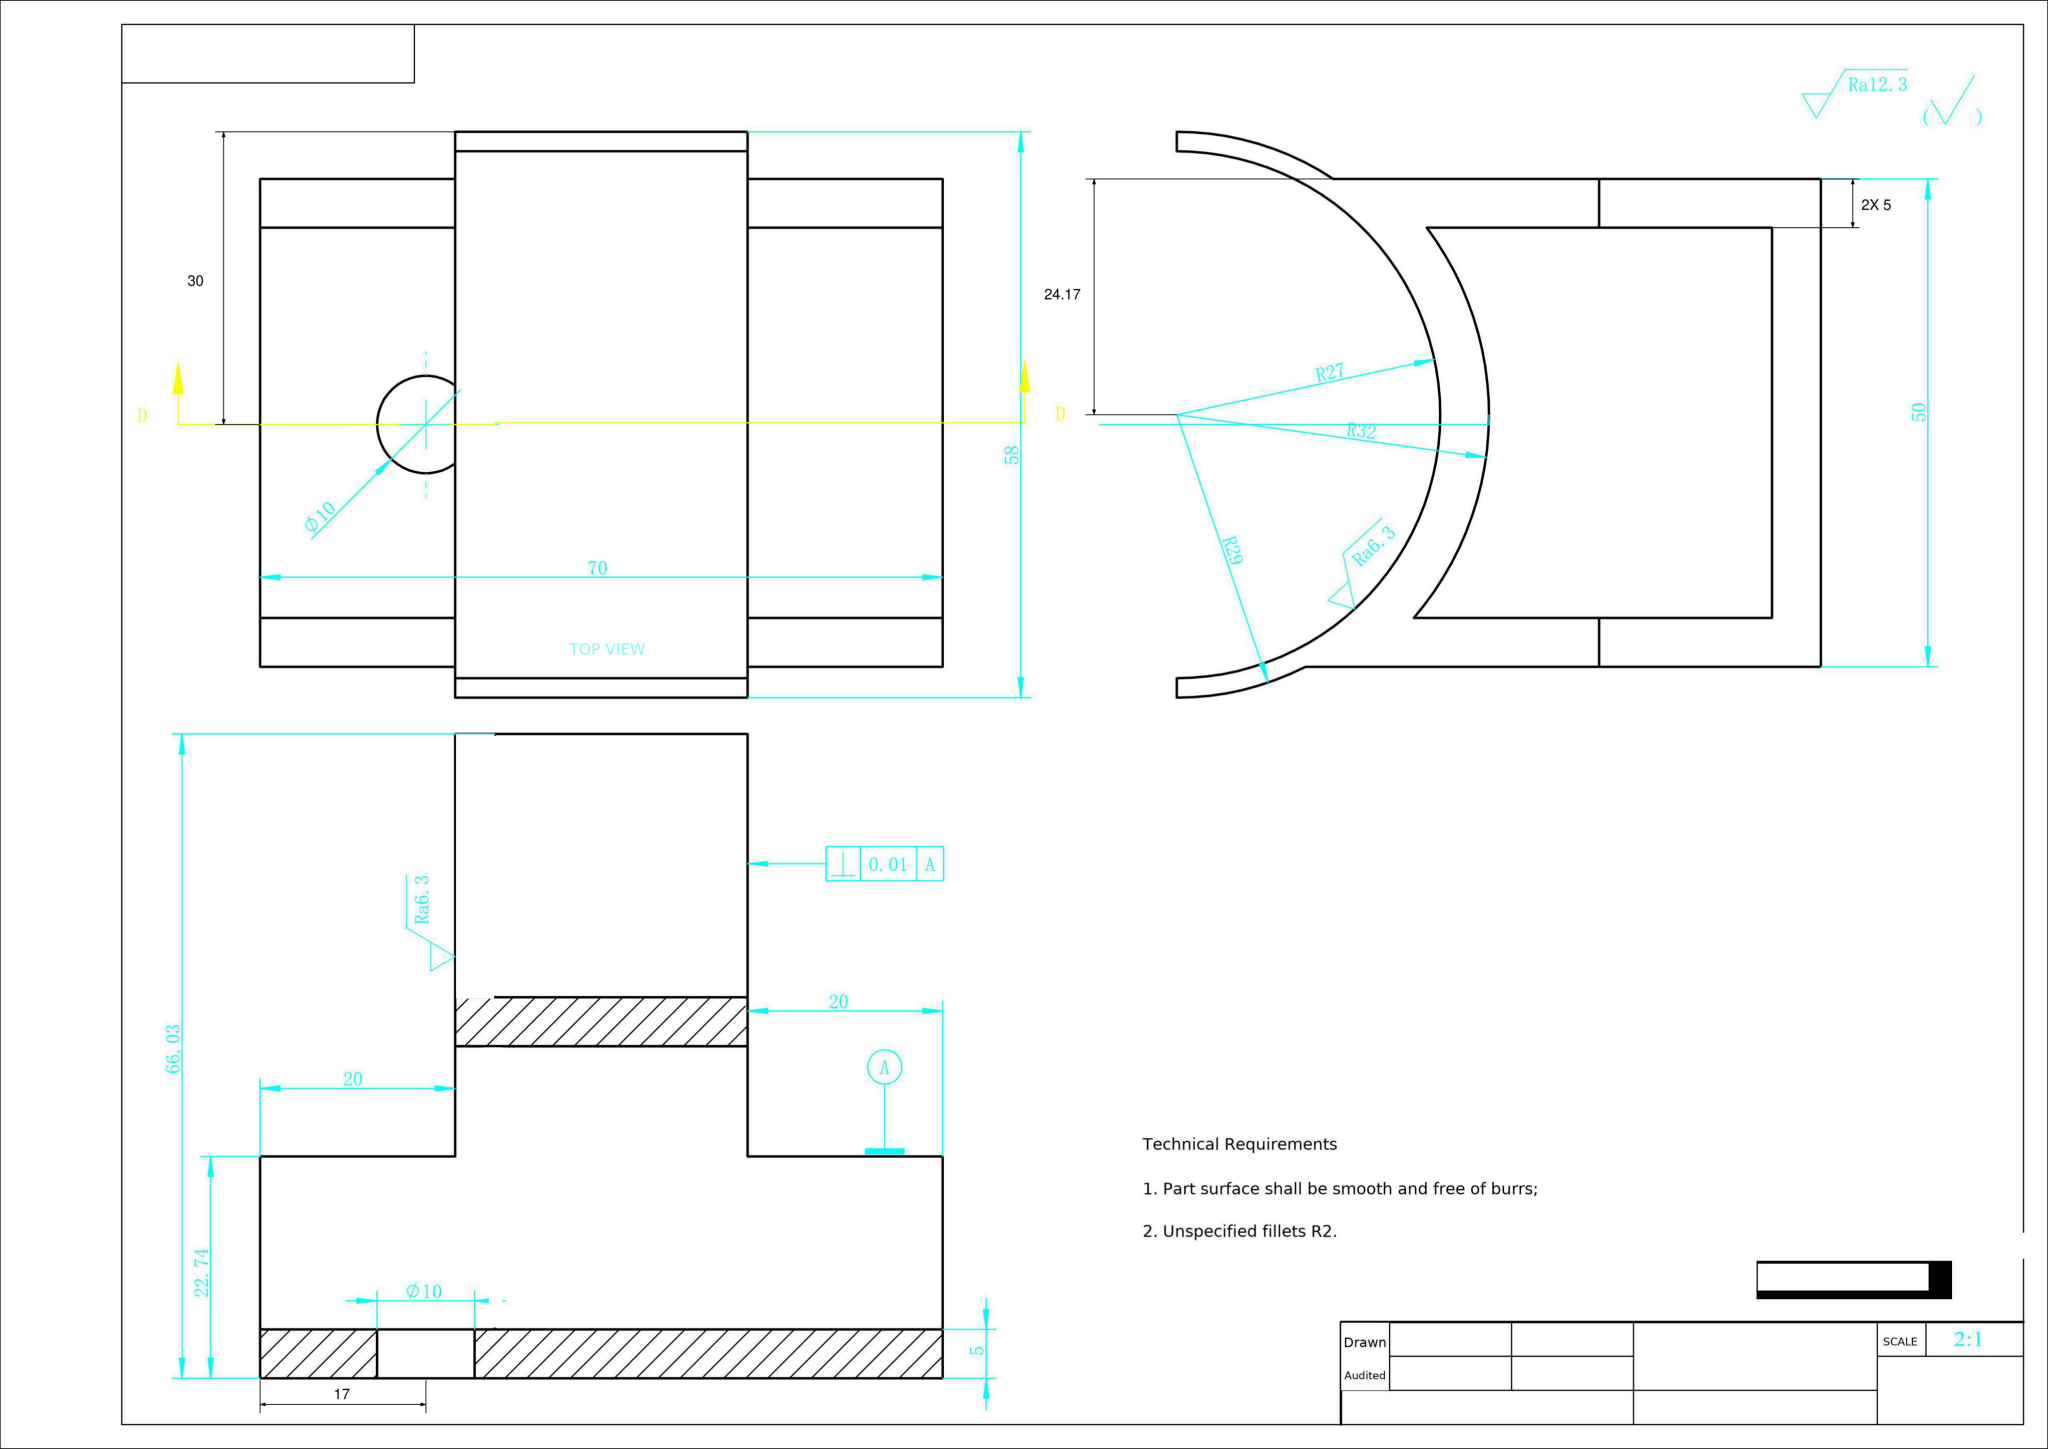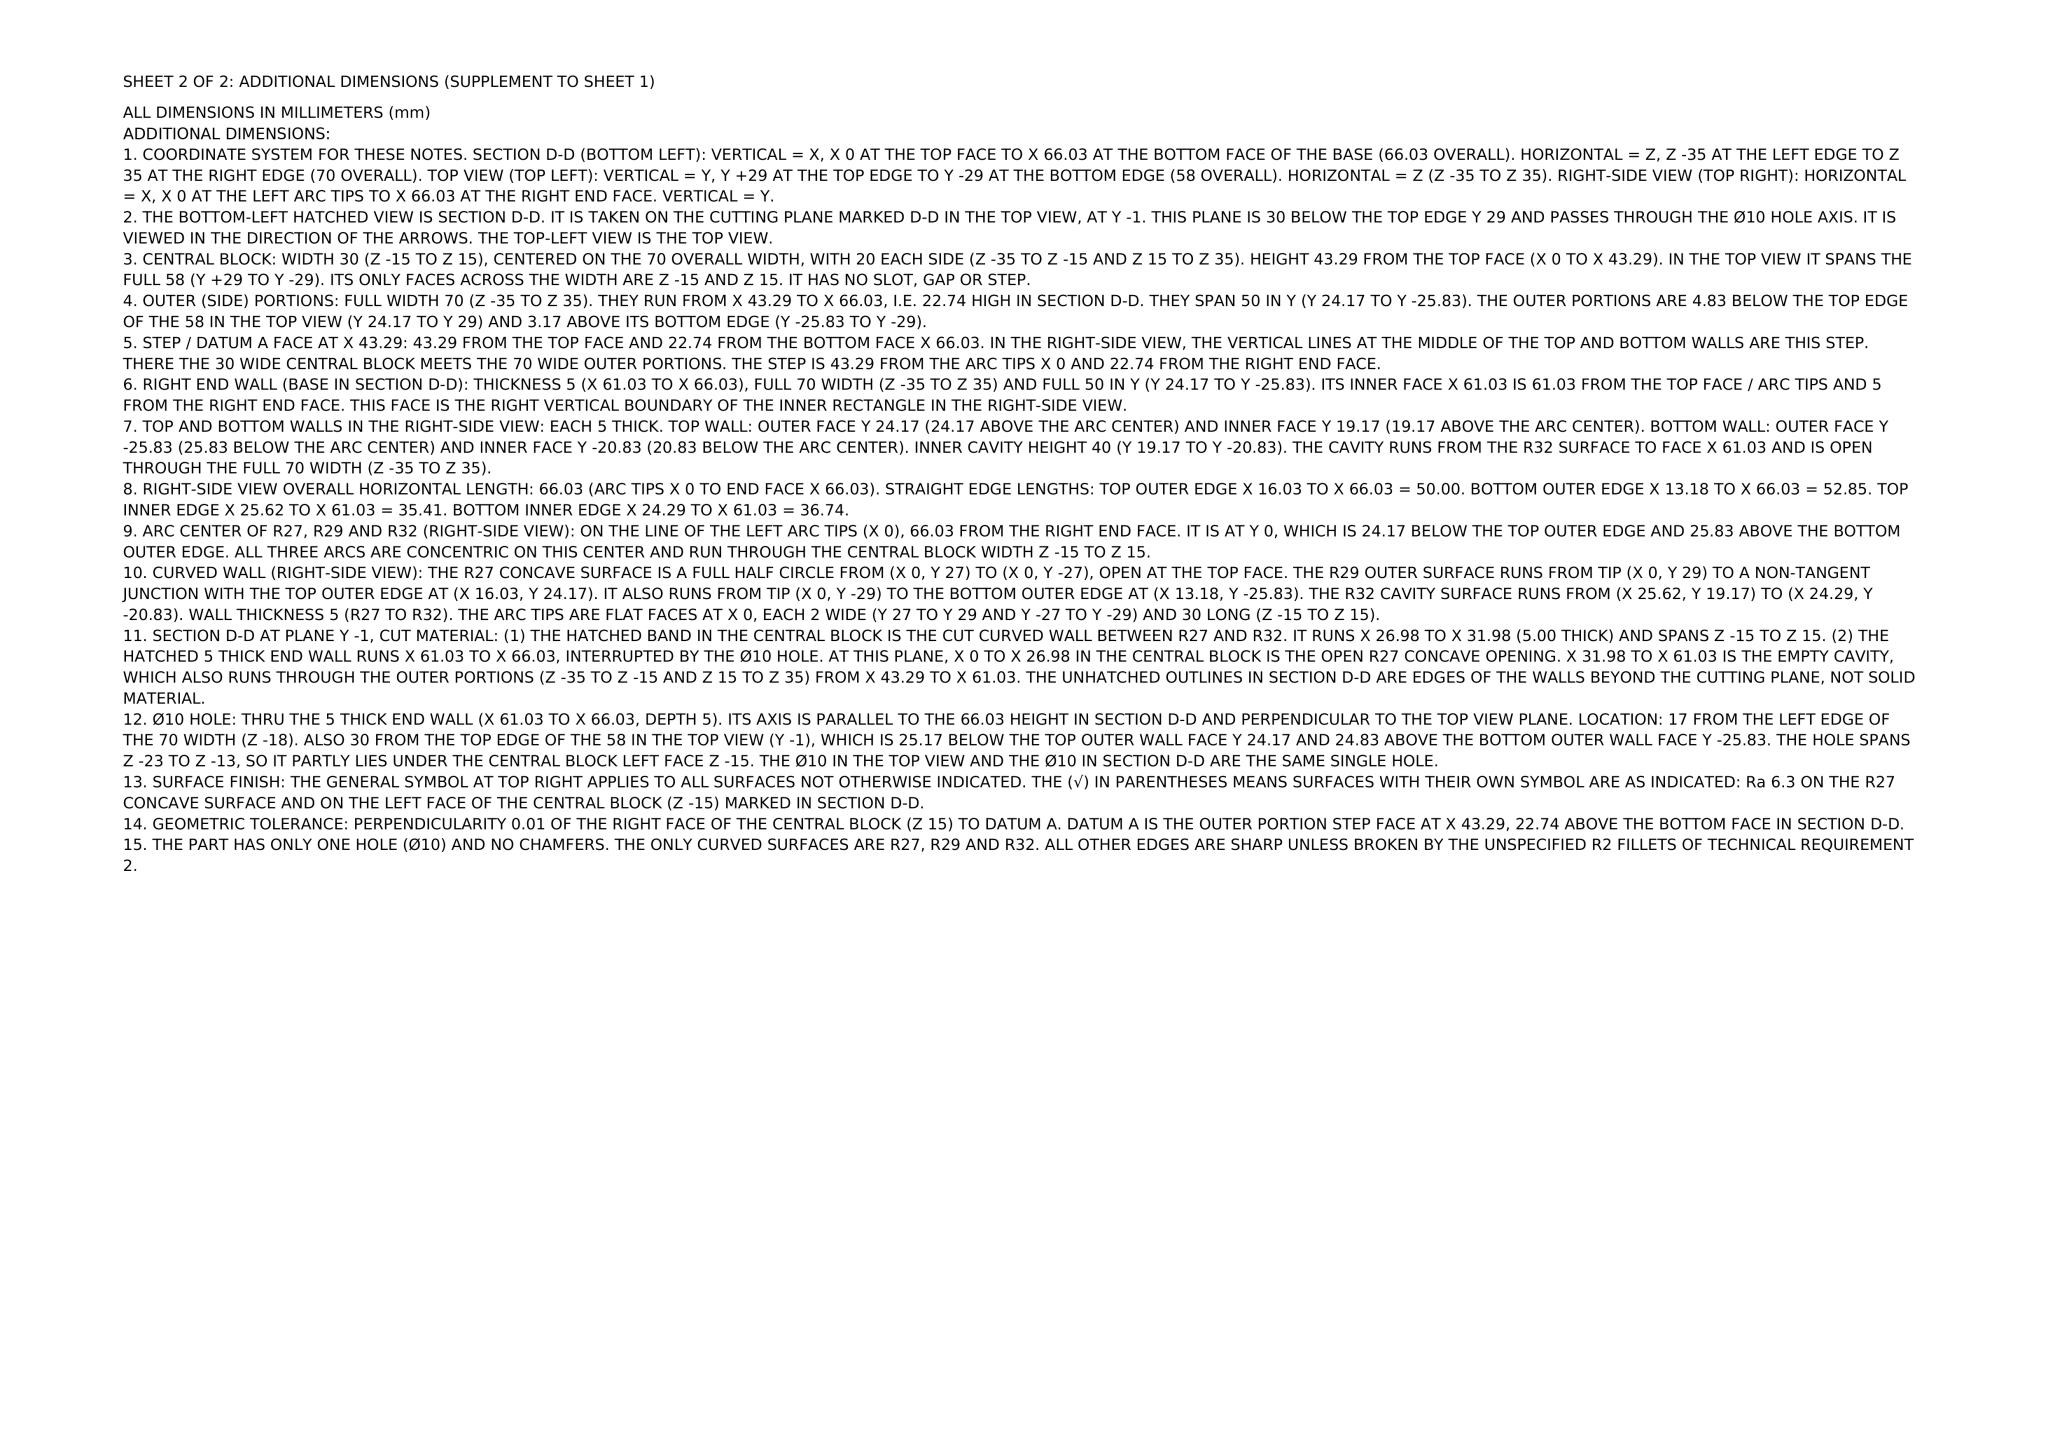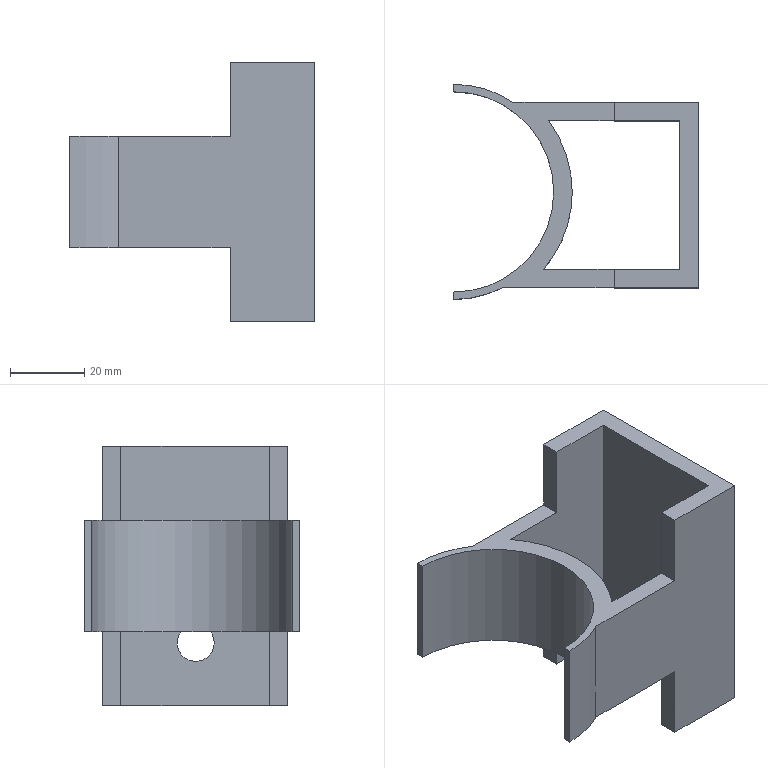Part | NX | mm | 1 solid | 23 faces | box 66.03 x 58 x 70 mm | volume 46292 mm3 | plane 16 | cylinder 7 | commonest cylinder face diameters 10 x2 64 x2 58 x2 54 x1
STEP:
#1=COLOUR_RGB('',0.7765,0.7569,0.7373);
#2=FILL_AREA_STYLE_COLOUR('',#1);
#3=FILL_AREA_STYLE('',(#2));
#4=SURFACE_STYLE_FILL_AREA(#3);
#5=SURFACE_SIDE_STYLE('',(#4));
#6=SURFACE_STYLE_USAGE(.BOTH.,#5);
#7=PRESENTATION_STYLE_ASSIGNMENT((#6));
#8=CARTESIAN_POINT('',(61.03,-6.,-18.));
#9=VERTEX_POINT('',#8);
#10=CARTESIAN_POINT('',(61.03,4.,-18.));
#11=VERTEX_POINT('',#10);
#12=CARTESIAN_POINT('',(61.03,-1.,-18.));
#13=DIRECTION('',(1.,0.,0.));
#14=DIRECTION('',(0.,0.,-1.));
#15=AXIS2_PLACEMENT_3D('',#12,#13,#14);
#16=CIRCLE('',#15,5.);
#17=EDGE_CURVE('',#9,#11,#16,.T.);
#18=ORIENTED_EDGE('',*,*,#17,.F.);
#19=CARTESIAN_POINT('',(66.03,-6.,-18.));
#20=VERTEX_POINT('',#19);
#21=CARTESIAN_POINT('',(56.03,-6.,-18.));
#22=DIRECTION('',(1.,0.,0.));
#23=VECTOR('',#22,1000.);
#24=LINE('',#21,#23);
#25=EDGE_CURVE('',#9,#20,#24,.T.);
#26=ORIENTED_EDGE('',*,*,#25,.T.);
#27=CARTESIAN_POINT('',(66.03,4.,-18.));
#28=VERTEX_POINT('',#27);
#29=CARTESIAN_POINT('',(66.03,-1.,-18.));
#30=DIRECTION('',(1.,0.,0.));
#31=DIRECTION('',(0.,1.,0.));
#32=AXIS2_PLACEMENT_3D('',#29,#30,#31);
#33=CIRCLE('',#32,5.);
#34=EDGE_CURVE('',#20,#28,#33,.T.);
#35=ORIENTED_EDGE('',*,*,#34,.T.);
#36=CARTESIAN_POINT('',(56.03,4.,-18.));
#37=DIRECTION('',(1.,0.,0.));
#38=VECTOR('',#37,1000.);
#39=LINE('',#36,#38);
#40=EDGE_CURVE('',#11,#28,#39,.T.);
#41=ORIENTED_EDGE('',*,*,#40,.F.);
#42=EDGE_LOOP('',(#18,#26,#35,#41));
#43=FACE_OUTER_BOUND('',#42,.T.);
#44=CARTESIAN_POINT('',(56.03,-1.,-18.));
#45=DIRECTION('',(1.,0.,0.));
#46=DIRECTION('',(0.,1.,0.));
#47=AXIS2_PLACEMENT_3D('',#44,#45,#46);
#48=CYLINDRICAL_SURFACE('',#47,5.);
#49=ADVANCED_FACE('',(#43),#48,.F.);
#50=CARTESIAN_POINT('',(24.289,-20.833,-15.));
#51=VERTEX_POINT('',#50);
#52=CARTESIAN_POINT('',(32.,-0.,-15.));
#53=VERTEX_POINT('',#52);
#54=CARTESIAN_POINT('',(0.,0.,-15.));
#55=DIRECTION('',(0.,0.,1.));
#56=DIRECTION('',(1.,0.,-0.));
#57=AXIS2_PLACEMENT_3D('',#54,#55,#56);
#58=CIRCLE('',#57,32.);
#59=EDGE_CURVE('',#51,#53,#58,.T.);
#60=ORIENTED_EDGE('',*,*,#59,.T.);
#61=CARTESIAN_POINT('',(32.,0.,15.));
#62=VERTEX_POINT('',#61);
#63=CARTESIAN_POINT('',(32.,0.,-35.));
#64=DIRECTION('',(0.,0.,1.));
#65=VECTOR('',#64,1000.);
#66=LINE('',#63,#65);
#67=EDGE_CURVE('',#53,#62,#66,.T.);
#68=ORIENTED_EDGE('',*,*,#67,.T.);
#69=CARTESIAN_POINT('',(24.289,-20.833,15.));
#70=VERTEX_POINT('',#69);
#71=CARTESIAN_POINT('',(0.,0.,15.));
#72=DIRECTION('',(-0.,-0.,-1.));
#73=DIRECTION('',(-1.,0.,0.));
#74=AXIS2_PLACEMENT_3D('',#71,#72,#73);
#75=CIRCLE('',#74,32.);
#76=EDGE_CURVE('',#62,#70,#75,.T.);
#77=ORIENTED_EDGE('',*,*,#76,.T.);
#78=CARTESIAN_POINT('',(24.289,-20.833,-35.));
#79=DIRECTION('',(0.,0.,1.));
#80=VECTOR('',#79,1000.);
#81=LINE('',#78,#80);
#82=EDGE_CURVE('',#51,#70,#81,.T.);
#83=ORIENTED_EDGE('',*,*,#82,.F.);
#84=EDGE_LOOP('',(#60,#68,#77,#83));
#85=FACE_OUTER_BOUND('',#84,.T.);
#86=CARTESIAN_POINT('',(0.,0.,-35.));
#87=DIRECTION('',(0.,0.,1.));
#88=DIRECTION('',(1.,0.,0.));
#89=AXIS2_PLACEMENT_3D('',#86,#87,#88);
#90=CYLINDRICAL_SURFACE('',#89,32.);
#91=ADVANCED_FACE('',(#85),#90,.T.);
#92=CARTESIAN_POINT('',(0.,29.,15.));
#93=VERTEX_POINT('',#92);
#94=CARTESIAN_POINT('',(0.,29.,-15.));
#95=VERTEX_POINT('',#94);
#96=CARTESIAN_POINT('',(0.,29.,35.));
#97=DIRECTION('',(0.,0.,-1.));
#98=VECTOR('',#97,1000.);
#99=LINE('',#96,#98);
#100=EDGE_CURVE('',#93,#95,#99,.T.);
#101=ORIENTED_EDGE('',*,*,#100,.F.);
#102=CARTESIAN_POINT('',(16.03,24.167,15.));
#103=VERTEX_POINT('',#102);
#104=CARTESIAN_POINT('',(0.,0.,15.));
#105=DIRECTION('',(-0.,-0.,-1.));
#106=DIRECTION('',(-1.,0.,0.));
#107=AXIS2_PLACEMENT_3D('',#104,#105,#106);
#108=CIRCLE('',#107,29.);
#109=EDGE_CURVE('',#93,#103,#108,.T.);
#110=ORIENTED_EDGE('',*,*,#109,.T.);
#111=CARTESIAN_POINT('',(16.03,24.167,-15.));
#112=VERTEX_POINT('',#111);
#113=CARTESIAN_POINT('',(16.03,24.167,35.));
#114=DIRECTION('',(0.,0.,-1.));
#115=VECTOR('',#114,1000.);
#116=LINE('',#113,#115);
#117=EDGE_CURVE('',#103,#112,#116,.T.);
#118=ORIENTED_EDGE('',*,*,#117,.T.);
#119=CARTESIAN_POINT('',(0.,0.,-15.));
#120=DIRECTION('',(0.,0.,1.));
#121=DIRECTION('',(1.,0.,-0.));
#122=AXIS2_PLACEMENT_3D('',#119,#120,#121);
#123=CIRCLE('',#122,29.);
#124=EDGE_CURVE('',#112,#95,#123,.T.);
#125=ORIENTED_EDGE('',*,*,#124,.T.);
#126=EDGE_LOOP('',(#101,#110,#118,#125));
#127=FACE_OUTER_BOUND('',#126,.T.);
#128=CARTESIAN_POINT('',(0.,0.,35.));
#129=DIRECTION('',(0.,0.,-1.));
#130=DIRECTION('',(-1.,0.,0.));
#131=AXIS2_PLACEMENT_3D('',#128,#129,#130);
#132=CYLINDRICAL_SURFACE('',#131,29.);
#133=ADVANCED_FACE('',(#127),#132,.T.);
#134=CARTESIAN_POINT('',(-0.,27.,15.));
#135=VERTEX_POINT('',#134);
#136=CARTESIAN_POINT('',(-0.,27.,-15.));
#137=VERTEX_POINT('',#136);
#138=CARTESIAN_POINT('',(0.,27.,35.));
#139=DIRECTION('',(0.,0.,-1.));
#140=VECTOR('',#139,1000.);
#141=LINE('',#138,#140);
#142=EDGE_CURVE('',#135,#137,#141,.T.);
#143=ORIENTED_EDGE('',*,*,#142,.F.);
#144=CARTESIAN_POINT('',(0.,29.,15.));
#145=DIRECTION('',(0.,1.,-0.));
#146=VECTOR('',#145,1000.);
#147=LINE('',#144,#146);
#148=EDGE_CURVE('',#135,#93,#147,.T.);
#149=ORIENTED_EDGE('',*,*,#148,.T.);
#150=ORIENTED_EDGE('',*,*,#100,.T.);
#151=CARTESIAN_POINT('',(0.,29.,-15.));
#152=DIRECTION('',(-0.,-1.,0.));
#153=VECTOR('',#152,1000.);
#154=LINE('',#151,#153);
#155=EDGE_CURVE('',#95,#137,#154,.T.);
#156=ORIENTED_EDGE('',*,*,#155,.T.);
#157=EDGE_LOOP('',(#143,#149,#150,#156));
#158=FACE_OUTER_BOUND('',#157,.T.);
#159=CARTESIAN_POINT('',(0.,29.,35.));
#160=DIRECTION('',(1.,-0.,0.));
#161=DIRECTION('',(0.,1.,0.));
#162=AXIS2_PLACEMENT_3D('',#159,#160,#161);
#163=PLANE('',#162);
#164=ADVANCED_FACE('',(#158),#163,.F.);
#165=CARTESIAN_POINT('',(-0.,-27.,15.));
#166=VERTEX_POINT('',#165);
#167=CARTESIAN_POINT('',(0.,-27.,-15.));
#168=VERTEX_POINT('',#167);
#169=CARTESIAN_POINT('',(0.,-27.,35.));
#170=DIRECTION('',(0.,0.,-1.));
#171=VECTOR('',#170,1000.);
#172=LINE('',#169,#171);
#173=EDGE_CURVE('',#166,#168,#172,.T.);
#174=ORIENTED_EDGE('',*,*,#173,.F.);
#175=CARTESIAN_POINT('',(0.,0.,15.));
#176=DIRECTION('',(0.,0.,1.));
#177=DIRECTION('',(-1.,0.,0.));
#178=AXIS2_PLACEMENT_3D('',#175,#176,#177);
#179=CIRCLE('',#178,27.);
#180=EDGE_CURVE('',#166,#135,#179,.T.);
#181=ORIENTED_EDGE('',*,*,#180,.T.);
#182=ORIENTED_EDGE('',*,*,#142,.T.);
#183=CARTESIAN_POINT('',(0.,0.,-15.));
#184=DIRECTION('',(-0.,-0.,-1.));
#185=DIRECTION('',(1.,0.,-0.));
#186=AXIS2_PLACEMENT_3D('',#183,#184,#185);
#187=CIRCLE('',#186,27.);
#188=EDGE_CURVE('',#137,#168,#187,.T.);
#189=ORIENTED_EDGE('',*,*,#188,.T.);
#190=EDGE_LOOP('',(#174,#181,#182,#189));
#191=FACE_OUTER_BOUND('',#190,.T.);
#192=CARTESIAN_POINT('',(0.,0.,35.));
#193=DIRECTION('',(0.,0.,-1.));
#194=DIRECTION('',(-1.,0.,0.));
#195=AXIS2_PLACEMENT_3D('',#192,#193,#194);
#196=CYLINDRICAL_SURFACE('',#195,27.);
#197=ADVANCED_FACE('',(#191),#196,.F.);
#198=CARTESIAN_POINT('',(0.,-29.,15.));
#199=VERTEX_POINT('',#198);
#200=CARTESIAN_POINT('',(0.,-29.,-15.));
#201=VERTEX_POINT('',#200);
#202=CARTESIAN_POINT('',(-0.,-29.,35.));
#203=DIRECTION('',(0.,0.,-1.));
#204=VECTOR('',#203,1000.);
#205=LINE('',#202,#204);
#206=EDGE_CURVE('',#199,#201,#205,.T.);
#207=ORIENTED_EDGE('',*,*,#206,.F.);
#208=CARTESIAN_POINT('',(-0.,-27.,15.));
#209=DIRECTION('',(-0.,1.,0.));
#210=VECTOR('',#209,1000.);
#211=LINE('',#208,#210);
#212=EDGE_CURVE('',#199,#166,#211,.T.);
#213=ORIENTED_EDGE('',*,*,#212,.T.);
#214=ORIENTED_EDGE('',*,*,#173,.T.);
#215=CARTESIAN_POINT('',(-0.,-27.,-15.));
#216=DIRECTION('',(0.,-1.,-0.));
#217=VECTOR('',#216,1000.);
#218=LINE('',#215,#217);
#219=EDGE_CURVE('',#168,#201,#218,.T.);
#220=ORIENTED_EDGE('',*,*,#219,.T.);
#221=EDGE_LOOP('',(#207,#213,#214,#220));
#222=FACE_OUTER_BOUND('',#221,.T.);
#223=CARTESIAN_POINT('',(0.,-27.,35.));
#224=DIRECTION('',(1.,0.,0.));
#225=DIRECTION('',(-0.,1.,0.));
#226=AXIS2_PLACEMENT_3D('',#223,#224,#225);
#227=PLANE('',#226);
#228=ADVANCED_FACE('',(#222),#227,.F.);
#229=CARTESIAN_POINT('',(13.177,-25.833,15.));
#230=VERTEX_POINT('',#229);
#231=CARTESIAN_POINT('',(13.177,-25.833,-15.));
#232=VERTEX_POINT('',#231);
#233=CARTESIAN_POINT('',(13.177,-25.833,35.));
#234=DIRECTION('',(0.,0.,-1.));
#235=VECTOR('',#234,1000.);
#236=LINE('',#233,#235);
#237=EDGE_CURVE('',#230,#232,#236,.T.);
#238=ORIENTED_EDGE('',*,*,#237,.F.);
#239=CARTESIAN_POINT('',(0.,0.,15.));
#240=DIRECTION('',(-0.,-0.,-1.));
#241=DIRECTION('',(-1.,0.,0.));
#242=AXIS2_PLACEMENT_3D('',#239,#240,#241);
#243=CIRCLE('',#242,29.);
#244=EDGE_CURVE('',#230,#199,#243,.T.);
#245=ORIENTED_EDGE('',*,*,#244,.T.);
#246=ORIENTED_EDGE('',*,*,#206,.T.);
#247=CARTESIAN_POINT('',(0.,0.,-15.));
#248=DIRECTION('',(0.,0.,1.));
#249=DIRECTION('',(1.,0.,-0.));
#250=AXIS2_PLACEMENT_3D('',#247,#248,#249);
#251=CIRCLE('',#250,29.);
#252=EDGE_CURVE('',#201,#232,#251,.T.);
#253=ORIENTED_EDGE('',*,*,#252,.T.);
#254=EDGE_LOOP('',(#238,#245,#246,#253));
#255=FACE_OUTER_BOUND('',#254,.T.);
#256=CARTESIAN_POINT('',(0.,0.,35.));
#257=DIRECTION('',(0.,0.,-1.));
#258=DIRECTION('',(-1.,0.,0.));
#259=AXIS2_PLACEMENT_3D('',#256,#257,#258);
#260=CYLINDRICAL_SURFACE('',#259,29.);
#261=ADVANCED_FACE('',(#255),#260,.T.);
#262=CARTESIAN_POINT('',(43.289,-25.833,35.));
#263=VERTEX_POINT('',#262);
#264=CARTESIAN_POINT('',(66.03,-25.833,35.));
#265=VERTEX_POINT('',#264);
#266=CARTESIAN_POINT('',(66.03,-25.833,35.));
#267=DIRECTION('',(1.,0.,0.));
#268=VECTOR('',#267,1000.);
#269=LINE('',#266,#268);
#270=EDGE_CURVE('',#263,#265,#269,.T.);
#271=ORIENTED_EDGE('',*,*,#270,.F.);
#272=CARTESIAN_POINT('',(43.289,-25.833,15.));
#273=VERTEX_POINT('',#272);
#274=CARTESIAN_POINT('',(43.289,-25.833,35.));
#275=DIRECTION('',(0.,0.,-1.));
#276=VECTOR('',#275,1000.);
#277=LINE('',#274,#276);
#278=EDGE_CURVE('',#263,#273,#277,.T.);
#279=ORIENTED_EDGE('',*,*,#278,.T.);
#280=CARTESIAN_POINT('',(66.03,-25.833,15.));
#281=DIRECTION('',(-1.,0.,0.));
#282=VECTOR('',#281,1000.);
#283=LINE('',#280,#282);
#284=EDGE_CURVE('',#273,#230,#283,.T.);
#285=ORIENTED_EDGE('',*,*,#284,.T.);
#286=ORIENTED_EDGE('',*,*,#237,.T.);
#287=CARTESIAN_POINT('',(43.289,-25.833,-15.));
#288=VERTEX_POINT('',#287);
#289=CARTESIAN_POINT('',(66.03,-25.833,-15.));
#290=DIRECTION('',(1.,0.,-0.));
#291=VECTOR('',#290,1000.);
#292=LINE('',#289,#291);
#293=EDGE_CURVE('',#232,#288,#292,.T.);
#294=ORIENTED_EDGE('',*,*,#293,.T.);
#295=CARTESIAN_POINT('',(43.289,-25.833,-35.));
#296=VERTEX_POINT('',#295);
#297=CARTESIAN_POINT('',(43.289,-25.833,35.));
#298=DIRECTION('',(0.,0.,-1.));
#299=VECTOR('',#298,1000.);
#300=LINE('',#297,#299);
#301=EDGE_CURVE('',#288,#296,#300,.T.);
#302=ORIENTED_EDGE('',*,*,#301,.T.);
#303=CARTESIAN_POINT('',(66.03,-25.833,-35.));
#304=VERTEX_POINT('',#303);
#305=CARTESIAN_POINT('',(66.03,-25.833,-35.));
#306=DIRECTION('',(1.,0.,0.));
#307=VECTOR('',#306,1000.);
#308=LINE('',#305,#307);
#309=EDGE_CURVE('',#296,#304,#308,.T.);
#310=ORIENTED_EDGE('',*,*,#309,.T.);
#311=CARTESIAN_POINT('',(66.03,-25.833,35.));
#312=DIRECTION('',(0.,0.,-1.));
#313=VECTOR('',#312,1000.);
#314=LINE('',#311,#313);
#315=EDGE_CURVE('',#265,#304,#314,.T.);
#316=ORIENTED_EDGE('',*,*,#315,.F.);
#317=EDGE_LOOP('',(#271,#279,#285,#286,#294,#302,#310,#316));
#318=FACE_OUTER_BOUND('',#317,.T.);
#319=CARTESIAN_POINT('',(66.03,-25.833,35.));
#320=DIRECTION('',(0.,1.,0.));
#321=DIRECTION('',(0.,0.,1.));
#322=AXIS2_PLACEMENT_3D('',#319,#320,#321);
#323=PLANE('',#322);
#324=ADVANCED_FACE('',(#318),#323,.F.);
#325=CARTESIAN_POINT('',(66.03,-1.,-18.));
#326=DIRECTION('',(1.,0.,0.));
#327=DIRECTION('',(0.,1.,0.));
#328=AXIS2_PLACEMENT_3D('',#325,#326,#327);
#329=CIRCLE('',#328,5.);
#330=EDGE_CURVE('',#28,#20,#329,.T.);
#331=ORIENTED_EDGE('',*,*,#330,.F.);
#332=ORIENTED_EDGE('',*,*,#34,.F.);
#333=EDGE_LOOP('',(#331,#332));
#334=FACE_BOUND('',#333,.T.);
#335=CARTESIAN_POINT('',(66.03,24.167,-35.));
#336=VERTEX_POINT('',#335);
#337=CARTESIAN_POINT('',(66.03,-25.833,-35.));
#338=DIRECTION('',(-0.,1.,0.));
#339=VECTOR('',#338,1000.);
#340=LINE('',#337,#339);
#341=EDGE_CURVE('',#304,#336,#340,.T.);
#342=ORIENTED_EDGE('',*,*,#341,.T.);
#343=CARTESIAN_POINT('',(66.03,24.167,35.));
#344=VERTEX_POINT('',#343);
#345=CARTESIAN_POINT('',(66.03,24.167,35.));
#346=DIRECTION('',(0.,0.,-1.));
#347=VECTOR('',#346,1000.);
#348=LINE('',#345,#347);
#349=EDGE_CURVE('',#344,#336,#348,.T.);
#350=ORIENTED_EDGE('',*,*,#349,.F.);
#351=CARTESIAN_POINT('',(66.03,-25.833,35.));
#352=DIRECTION('',(-0.,1.,0.));
#353=VECTOR('',#352,1000.);
#354=LINE('',#351,#353);
#355=EDGE_CURVE('',#265,#344,#354,.T.);
#356=ORIENTED_EDGE('',*,*,#355,.F.);
#357=ORIENTED_EDGE('',*,*,#315,.T.);
#358=EDGE_LOOP('',(#342,#350,#356,#357));
#359=FACE_OUTER_BOUND('',#358,.T.);
#360=CARTESIAN_POINT('',(66.03,-25.833,35.));
#361=DIRECTION('',(-1.,-0.,0.));
#362=DIRECTION('',(0.,-1.,0.));
#363=AXIS2_PLACEMENT_3D('',#360,#361,#362);
#364=PLANE('',#363);
#365=ADVANCED_FACE('',(#334,#359),#364,.F.);
#366=CARTESIAN_POINT('',(43.289,24.167,15.));
#367=VERTEX_POINT('',#366);
#368=CARTESIAN_POINT('',(66.03,24.167,15.));
#369=DIRECTION('',(1.,0.,-0.));
#370=VECTOR('',#369,1000.);
#371=LINE('',#368,#370);
#372=EDGE_CURVE('',#103,#367,#371,.T.);
#373=ORIENTED_EDGE('',*,*,#372,.T.);
#374=CARTESIAN_POINT('',(43.289,24.167,35.));
#375=VERTEX_POINT('',#374);
#376=CARTESIAN_POINT('',(43.289,24.167,35.));
#377=DIRECTION('',(0.,0.,1.));
#378=VECTOR('',#377,1000.);
#379=LINE('',#376,#378);
#380=EDGE_CURVE('',#367,#375,#379,.T.);
#381=ORIENTED_EDGE('',*,*,#380,.T.);
#382=CARTESIAN_POINT('',(66.03,24.167,35.));
#383=DIRECTION('',(-1.,-0.,0.));
#384=VECTOR('',#383,1000.);
#385=LINE('',#382,#384);
#386=EDGE_CURVE('',#344,#375,#385,.T.);
#387=ORIENTED_EDGE('',*,*,#386,.F.);
#388=ORIENTED_EDGE('',*,*,#349,.T.);
#389=CARTESIAN_POINT('',(43.289,24.167,-35.));
#390=VERTEX_POINT('',#389);
#391=CARTESIAN_POINT('',(66.03,24.167,-35.));
#392=DIRECTION('',(-1.,-0.,0.));
#393=VECTOR('',#392,1000.);
#394=LINE('',#391,#393);
#395=EDGE_CURVE('',#336,#390,#394,.T.);
#396=ORIENTED_EDGE('',*,*,#395,.T.);
#397=CARTESIAN_POINT('',(43.289,24.167,-15.));
#398=VERTEX_POINT('',#397);
#399=CARTESIAN_POINT('',(43.289,24.167,35.));
#400=DIRECTION('',(0.,0.,1.));
#401=VECTOR('',#400,1000.);
#402=LINE('',#399,#401);
#403=EDGE_CURVE('',#390,#398,#402,.T.);
#404=ORIENTED_EDGE('',*,*,#403,.T.);
#405=CARTESIAN_POINT('',(66.03,24.167,-15.));
#406=DIRECTION('',(-1.,-0.,0.));
#407=VECTOR('',#406,1000.);
#408=LINE('',#405,#407);
#409=EDGE_CURVE('',#398,#112,#408,.T.);
#410=ORIENTED_EDGE('',*,*,#409,.T.);
#411=ORIENTED_EDGE('',*,*,#117,.F.);
#412=EDGE_LOOP('',(#373,#381,#387,#388,#396,#404,#410,#411));
#413=FACE_OUTER_BOUND('',#412,.T.);
#414=CARTESIAN_POINT('',(66.03,24.167,35.));
#415=DIRECTION('',(0.,-1.,0.));
#416=DIRECTION('',(1.,0.,0.));
#417=AXIS2_PLACEMENT_3D('',#414,#415,#416);
#418=PLANE('',#417);
#419=ADVANCED_FACE('',(#413),#418,.F.);
#420=CARTESIAN_POINT('',(43.289,-20.833,35.));
#421=VERTEX_POINT('',#420);
#422=CARTESIAN_POINT('',(43.289,0.,35.));
#423=DIRECTION('',(-0.,1.,0.));
#424=VECTOR('',#423,1000.);
#425=LINE('',#422,#424);
#426=EDGE_CURVE('',#263,#421,#425,.T.);
#427=ORIENTED_EDGE('',*,*,#426,.F.);
#428=ORIENTED_EDGE('',*,*,#270,.T.);
#429=ORIENTED_EDGE('',*,*,#355,.T.);
#430=ORIENTED_EDGE('',*,*,#386,.T.);
#431=CARTESIAN_POINT('',(43.289,19.167,35.));
#432=VERTEX_POINT('',#431);
#433=CARTESIAN_POINT('',(43.289,0.,35.));
#434=DIRECTION('',(-0.,1.,0.));
#435=VECTOR('',#434,1000.);
#436=LINE('',#433,#435);
#437=EDGE_CURVE('',#432,#375,#436,.T.);
#438=ORIENTED_EDGE('',*,*,#437,.F.);
#439=CARTESIAN_POINT('',(61.03,19.167,35.));
#440=VERTEX_POINT('',#439);
#441=CARTESIAN_POINT('',(61.03,19.167,35.));
#442=DIRECTION('',(-1.,0.,0.));
#443=VECTOR('',#442,1000.);
#444=LINE('',#441,#443);
#445=EDGE_CURVE('',#440,#432,#444,.T.);
#446=ORIENTED_EDGE('',*,*,#445,.F.);
#447=CARTESIAN_POINT('',(61.03,-20.833,35.));
#448=VERTEX_POINT('',#447);
#449=CARTESIAN_POINT('',(61.03,-20.833,35.));
#450=DIRECTION('',(0.,1.,0.));
#451=VECTOR('',#450,1000.);
#452=LINE('',#449,#451);
#453=EDGE_CURVE('',#448,#440,#452,.T.);
#454=ORIENTED_EDGE('',*,*,#453,.F.);
#455=CARTESIAN_POINT('',(24.289,-20.833,35.));
#456=DIRECTION('',(1.,0.,0.));
#457=VECTOR('',#456,1000.);
#458=LINE('',#455,#457);
#459=EDGE_CURVE('',#421,#448,#458,.T.);
#460=ORIENTED_EDGE('',*,*,#459,.F.);
#461=EDGE_LOOP('',(#427,#428,#429,#430,#438,#446,#454,#460));
#462=FACE_OUTER_BOUND('',#461,.T.);
#463=CARTESIAN_POINT('',(0.,0.,35.));
#464=DIRECTION('',(0.,0.,1.));
#465=DIRECTION('',(1.,0.,0.));
#466=AXIS2_PLACEMENT_3D('',#463,#464,#465);
#467=PLANE('',#466);
#468=ADVANCED_FACE('',(#462),#467,.T.);
#469=ORIENTED_EDGE('',*,*,#309,.F.);
#470=CARTESIAN_POINT('',(43.289,-20.833,-35.));
#471=VERTEX_POINT('',#470);
#472=CARTESIAN_POINT('',(43.289,0.,-35.));
#473=DIRECTION('',(-0.,1.,0.));
#474=VECTOR('',#473,1000.);
#475=LINE('',#472,#474);
#476=EDGE_CURVE('',#296,#471,#475,.T.);
#477=ORIENTED_EDGE('',*,*,#476,.T.);
#478=CARTESIAN_POINT('',(61.03,-20.833,-35.));
#479=VERTEX_POINT('',#478);
#480=CARTESIAN_POINT('',(24.289,-20.833,-35.));
#481=DIRECTION('',(1.,0.,0.));
#482=VECTOR('',#481,1000.);
#483=LINE('',#480,#482);
#484=EDGE_CURVE('',#471,#479,#483,.T.);
#485=ORIENTED_EDGE('',*,*,#484,.T.);
#486=CARTESIAN_POINT('',(61.03,19.167,-35.));
#487=VERTEX_POINT('',#486);
#488=CARTESIAN_POINT('',(61.03,-20.833,-35.));
#489=DIRECTION('',(0.,1.,0.));
#490=VECTOR('',#489,1000.);
#491=LINE('',#488,#490);
#492=EDGE_CURVE('',#479,#487,#491,.T.);
#493=ORIENTED_EDGE('',*,*,#492,.T.);
#494=CARTESIAN_POINT('',(43.289,19.167,-35.));
#495=VERTEX_POINT('',#494);
#496=CARTESIAN_POINT('',(61.03,19.167,-35.));
#497=DIRECTION('',(-1.,0.,0.));
#498=VECTOR('',#497,1000.);
#499=LINE('',#496,#498);
#500=EDGE_CURVE('',#487,#495,#499,.T.);
#501=ORIENTED_EDGE('',*,*,#500,.T.);
#502=CARTESIAN_POINT('',(43.289,0.,-35.));
#503=DIRECTION('',(-0.,1.,0.));
#504=VECTOR('',#503,1000.);
#505=LINE('',#502,#504);
#506=EDGE_CURVE('',#495,#390,#505,.T.);
#507=ORIENTED_EDGE('',*,*,#506,.T.);
#508=ORIENTED_EDGE('',*,*,#395,.F.);
#509=ORIENTED_EDGE('',*,*,#341,.F.);
#510=EDGE_LOOP('',(#469,#477,#485,#493,#501,#507,#508,#509));
#511=FACE_OUTER_BOUND('',#510,.T.);
#512=CARTESIAN_POINT('',(0.,0.,-35.));
#513=DIRECTION('',(0.,0.,1.));
#514=DIRECTION('',(1.,0.,0.));
#515=AXIS2_PLACEMENT_3D('',#512,#513,#514);
#516=PLANE('',#515);
#517=ADVANCED_FACE('',(#511),#516,.F.);
#518=CARTESIAN_POINT('',(61.03,-1.,-18.));
#519=DIRECTION('',(1.,0.,0.));
#520=DIRECTION('',(0.,0.,-1.));
#521=AXIS2_PLACEMENT_3D('',#518,#519,#520);
#522=CIRCLE('',#521,5.);
#523=EDGE_CURVE('',#11,#9,#522,.T.);
#524=ORIENTED_EDGE('',*,*,#523,.T.);
#525=ORIENTED_EDGE('',*,*,#17,.T.);
#526=EDGE_LOOP('',(#524,#525));
#527=FACE_BOUND('',#526,.T.);
#528=ORIENTED_EDGE('',*,*,#453,.T.);
#529=CARTESIAN_POINT('',(61.03,19.167,-35.));
#530=DIRECTION('',(0.,0.,1.));
#531=VECTOR('',#530,1000.);
#532=LINE('',#529,#531);
#533=EDGE_CURVE('',#487,#440,#532,.T.);
#534=ORIENTED_EDGE('',*,*,#533,.F.);
#535=ORIENTED_EDGE('',*,*,#492,.F.);
#536=CARTESIAN_POINT('',(61.03,-20.833,-35.));
#537=DIRECTION('',(0.,0.,1.));
#538=VECTOR('',#537,1000.);
#539=LINE('',#536,#538);
#540=EDGE_CURVE('',#479,#448,#539,.T.);
#541=ORIENTED_EDGE('',*,*,#540,.T.);
#542=EDGE_LOOP('',(#528,#534,#535,#541));
#543=FACE_OUTER_BOUND('',#542,.T.);
#544=CARTESIAN_POINT('',(61.03,-20.833,-35.));
#545=DIRECTION('',(1.,0.,0.));
#546=DIRECTION('',(0.,0.,-1.));
#547=AXIS2_PLACEMENT_3D('',#544,#545,#546);
#548=PLANE('',#547);
#549=ADVANCED_FACE('',(#527,#543),#548,.F.);
#550=CARTESIAN_POINT('',(43.289,-20.833,15.));
#551=VERTEX_POINT('',#550);
#552=CARTESIAN_POINT('',(24.289,-20.833,15.));
#553=DIRECTION('',(1.,0.,-0.));
#554=VECTOR('',#553,1000.);
#555=LINE('',#552,#554);
#556=EDGE_CURVE('',#70,#551,#555,.T.);
#557=ORIENTED_EDGE('',*,*,#556,.T.);
#558=CARTESIAN_POINT('',(43.289,-20.833,-35.));
#559=DIRECTION('',(0.,0.,1.));
#560=VECTOR('',#559,1000.);
#561=LINE('',#558,#560);
#562=EDGE_CURVE('',#551,#421,#561,.T.);
#563=ORIENTED_EDGE('',*,*,#562,.T.);
#564=ORIENTED_EDGE('',*,*,#459,.T.);
#565=ORIENTED_EDGE('',*,*,#540,.F.);
#566=ORIENTED_EDGE('',*,*,#484,.F.);
#567=CARTESIAN_POINT('',(43.289,-20.833,-15.));
#568=VERTEX_POINT('',#567);
#569=CARTESIAN_POINT('',(43.289,-20.833,-35.));
#570=DIRECTION('',(0.,0.,1.));
#571=VECTOR('',#570,1000.);
#572=LINE('',#569,#571);
#573=EDGE_CURVE('',#471,#568,#572,.T.);
#574=ORIENTED_EDGE('',*,*,#573,.T.);
#575=CARTESIAN_POINT('',(24.289,-20.833,-15.));
#576=DIRECTION('',(-1.,0.,0.));
#577=VECTOR('',#576,1000.);
#578=LINE('',#575,#577);
#579=EDGE_CURVE('',#568,#51,#578,.T.);
#580=ORIENTED_EDGE('',*,*,#579,.T.);
#581=ORIENTED_EDGE('',*,*,#82,.T.);
#582=EDGE_LOOP('',(#557,#563,#564,#565,#566,#574,#580,#581));
#583=FACE_OUTER_BOUND('',#582,.T.);
#584=CARTESIAN_POINT('',(24.289,-20.833,-35.));
#585=DIRECTION('',(0.,-1.,0.));
#586=DIRECTION('',(0.,0.,-1.));
#587=AXIS2_PLACEMENT_3D('',#584,#585,#586);
#588=PLANE('',#587);
#589=ADVANCED_FACE('',(#583),#588,.F.);
#590=ORIENTED_EDGE('',*,*,#67,.F.);
#591=CARTESIAN_POINT('',(25.625,19.167,-15.));
#592=VERTEX_POINT('',#591);
#593=CARTESIAN_POINT('',(0.,0.,-15.));
#594=DIRECTION('',(0.,0.,1.));
#595=DIRECTION('',(1.,0.,-0.));
#596=AXIS2_PLACEMENT_3D('',#593,#594,#595);
#597=CIRCLE('',#596,32.);
#598=EDGE_CURVE('',#53,#592,#597,.T.);
#599=ORIENTED_EDGE('',*,*,#598,.T.);
#600=CARTESIAN_POINT('',(25.625,19.167,15.));
#601=VERTEX_POINT('',#600);
#602=CARTESIAN_POINT('',(25.625,19.167,-35.));
#603=DIRECTION('',(0.,0.,1.));
#604=VECTOR('',#603,1000.);
#605=LINE('',#602,#604);
#606=EDGE_CURVE('',#592,#601,#605,.T.);
#607=ORIENTED_EDGE('',*,*,#606,.T.);
#608=CARTESIAN_POINT('',(0.,0.,15.));
#609=DIRECTION('',(-0.,-0.,-1.));
#610=DIRECTION('',(-1.,0.,0.));
#611=AXIS2_PLACEMENT_3D('',#608,#609,#610);
#612=CIRCLE('',#611,32.);
#613=EDGE_CURVE('',#601,#62,#612,.T.);
#614=ORIENTED_EDGE('',*,*,#613,.T.);
#615=EDGE_LOOP('',(#590,#599,#607,#614));
#616=FACE_OUTER_BOUND('',#615,.T.);
#617=CARTESIAN_POINT('',(0.,0.,-35.));
#618=DIRECTION('',(0.,0.,1.));
#619=DIRECTION('',(1.,0.,0.));
#620=AXIS2_PLACEMENT_3D('',#617,#618,#619);
#621=CYLINDRICAL_SURFACE('',#620,32.);
#622=ADVANCED_FACE('',(#616),#621,.T.);
#623=ORIENTED_EDGE('',*,*,#445,.T.);
#624=CARTESIAN_POINT('',(43.289,19.167,15.));
#625=VERTEX_POINT('',#624);
#626=CARTESIAN_POINT('',(43.289,19.167,-35.));
#627=DIRECTION('',(0.,0.,-1.));
#628=VECTOR('',#627,1000.);
#629=LINE('',#626,#628);
#630=EDGE_CURVE('',#432,#625,#629,.T.);
#631=ORIENTED_EDGE('',*,*,#630,.T.);
#632=CARTESIAN_POINT('',(61.03,19.167,15.));
#633=DIRECTION('',(-1.,0.,0.));
#634=VECTOR('',#633,1000.);
#635=LINE('',#632,#634);
#636=EDGE_CURVE('',#625,#601,#635,.T.);
#637=ORIENTED_EDGE('',*,*,#636,.T.);
#638=ORIENTED_EDGE('',*,*,#606,.F.);
#639=CARTESIAN_POINT('',(43.289,19.167,-15.));
#640=VERTEX_POINT('',#639);
#641=CARTESIAN_POINT('',(61.03,19.167,-15.));
#642=DIRECTION('',(1.,0.,-0.));
#643=VECTOR('',#642,1000.);
#644=LINE('',#641,#643);
#645=EDGE_CURVE('',#592,#640,#644,.T.);
#646=ORIENTED_EDGE('',*,*,#645,.T.);
#647=CARTESIAN_POINT('',(43.289,19.167,-35.));
#648=DIRECTION('',(0.,0.,-1.));
#649=VECTOR('',#648,1000.);
#650=LINE('',#647,#649);
#651=EDGE_CURVE('',#640,#495,#650,.T.);
#652=ORIENTED_EDGE('',*,*,#651,.T.);
#653=ORIENTED_EDGE('',*,*,#500,.F.);
#654=ORIENTED_EDGE('',*,*,#533,.T.);
#655=EDGE_LOOP('',(#623,#631,#637,#638,#646,#652,#653,#654));
#656=FACE_OUTER_BOUND('',#655,.T.);
#657=CARTESIAN_POINT('',(61.03,19.167,-35.));
#658=DIRECTION('',(0.,1.,0.));
#659=DIRECTION('',(0.,0.,1.));
#660=AXIS2_PLACEMENT_3D('',#657,#658,#659);
#661=PLANE('',#660);
#662=ADVANCED_FACE('',(#656),#661,.F.);
#663=ORIENTED_EDGE('',*,*,#25,.F.);
#664=ORIENTED_EDGE('',*,*,#523,.F.);
#665=ORIENTED_EDGE('',*,*,#40,.T.);
#666=ORIENTED_EDGE('',*,*,#330,.T.);
#667=EDGE_LOOP('',(#663,#664,#665,#666));
#668=FACE_OUTER_BOUND('',#667,.T.);
#669=CARTESIAN_POINT('',(56.03,-1.,-18.));
#670=DIRECTION('',(1.,0.,0.));
#671=DIRECTION('',(0.,1.,0.));
#672=AXIS2_PLACEMENT_3D('',#669,#670,#671);
#673=CYLINDRICAL_SURFACE('',#672,5.);
#674=ADVANCED_FACE('',(#668),#673,.F.);
#675=ORIENTED_EDGE('',*,*,#252,.F.);
#676=ORIENTED_EDGE('',*,*,#219,.F.);
#677=ORIENTED_EDGE('',*,*,#188,.F.);
#678=ORIENTED_EDGE('',*,*,#155,.F.);
#679=ORIENTED_EDGE('',*,*,#124,.F.);
#680=ORIENTED_EDGE('',*,*,#409,.F.);
#681=CARTESIAN_POINT('',(43.289,-35.833,-15.));
#682=DIRECTION('',(-0.,1.,0.));
#683=VECTOR('',#682,1000.);
#684=LINE('',#681,#683);
#685=EDGE_CURVE('',#640,#398,#684,.T.);
#686=ORIENTED_EDGE('',*,*,#685,.F.);
#687=ORIENTED_EDGE('',*,*,#645,.F.);
#688=ORIENTED_EDGE('',*,*,#598,.F.);
#689=ORIENTED_EDGE('',*,*,#59,.F.);
#690=ORIENTED_EDGE('',*,*,#579,.F.);
#691=CARTESIAN_POINT('',(43.289,-35.833,-15.));
#692=DIRECTION('',(-0.,1.,0.));
#693=VECTOR('',#692,1000.);
#694=LINE('',#691,#693);
#695=EDGE_CURVE('',#288,#568,#694,.T.);
#696=ORIENTED_EDGE('',*,*,#695,.F.);
#697=ORIENTED_EDGE('',*,*,#293,.F.);
#698=EDGE_LOOP('',(#675,#676,#677,#678,#679,#680,#686,#687,#688,#689,#690,#696,#697));
#699=FACE_OUTER_BOUND('',#698,.T.);
#700=CARTESIAN_POINT('',(43.289,-35.833,-15.));
#701=DIRECTION('',(0.,0.,1.));
#702=DIRECTION('',(1.,0.,-0.));
#703=AXIS2_PLACEMENT_3D('',#700,#701,#702);
#704=PLANE('',#703);
#705=ADVANCED_FACE('',(#699),#704,.F.);
#706=ORIENTED_EDGE('',*,*,#695,.T.);
#707=ORIENTED_EDGE('',*,*,#573,.F.);
#708=ORIENTED_EDGE('',*,*,#476,.F.);
#709=ORIENTED_EDGE('',*,*,#301,.F.);
#710=EDGE_LOOP('',(#706,#707,#708,#709));
#711=FACE_OUTER_BOUND('',#710,.T.);
#712=CARTESIAN_POINT('',(43.289,-35.833,-42.21));
#713=DIRECTION('',(1.,0.,0.));
#714=DIRECTION('',(-0.,1.,0.));
#715=AXIS2_PLACEMENT_3D('',#712,#713,#714);
#716=PLANE('',#715);
#717=ADVANCED_FACE('',(#711),#716,.F.);
#718=ORIENTED_EDGE('',*,*,#506,.F.);
#719=ORIENTED_EDGE('',*,*,#651,.F.);
#720=ORIENTED_EDGE('',*,*,#685,.T.);
#721=ORIENTED_EDGE('',*,*,#403,.F.);
#722=EDGE_LOOP('',(#718,#719,#720,#721));
#723=FACE_OUTER_BOUND('',#722,.T.);
#724=CARTESIAN_POINT('',(43.289,-35.833,-42.21));
#725=DIRECTION('',(1.,0.,0.));
#726=DIRECTION('',(-0.,1.,0.));
#727=AXIS2_PLACEMENT_3D('',#724,#725,#726);
#728=PLANE('',#727);
#729=ADVANCED_FACE('',(#723),#728,.F.);
#730=ORIENTED_EDGE('',*,*,#426,.T.);
#731=ORIENTED_EDGE('',*,*,#562,.F.);
#732=CARTESIAN_POINT('',(43.289,-35.833,15.));
#733=DIRECTION('',(-0.,1.,0.));
#734=VECTOR('',#733,1000.);
#735=LINE('',#732,#734);
#736=EDGE_CURVE('',#273,#551,#735,.T.);
#737=ORIENTED_EDGE('',*,*,#736,.F.);
#738=ORIENTED_EDGE('',*,*,#278,.F.);
#739=EDGE_LOOP('',(#730,#731,#737,#738));
#740=FACE_OUTER_BOUND('',#739,.T.);
#741=CARTESIAN_POINT('',(43.289,-35.833,42.21));
#742=DIRECTION('',(1.,0.,0.));
#743=DIRECTION('',(-0.,1.,0.));
#744=AXIS2_PLACEMENT_3D('',#741,#742,#743);
#745=PLANE('',#744);
#746=ADVANCED_FACE('',(#740),#745,.F.);
#747=CARTESIAN_POINT('',(43.289,-35.833,15.));
#748=DIRECTION('',(-0.,1.,0.));
#749=VECTOR('',#748,1000.);
#750=LINE('',#747,#749);
#751=EDGE_CURVE('',#625,#367,#750,.T.);
#752=ORIENTED_EDGE('',*,*,#751,.F.);
#753=ORIENTED_EDGE('',*,*,#630,.F.);
#754=ORIENTED_EDGE('',*,*,#437,.T.);
#755=ORIENTED_EDGE('',*,*,#380,.F.);
#756=EDGE_LOOP('',(#752,#753,#754,#755));
#757=FACE_OUTER_BOUND('',#756,.T.);
#758=CARTESIAN_POINT('',(43.289,-35.833,42.21));
#759=DIRECTION('',(1.,0.,0.));
#760=DIRECTION('',(-0.,1.,0.));
#761=AXIS2_PLACEMENT_3D('',#758,#759,#760);
#762=PLANE('',#761);
#763=ADVANCED_FACE('',(#757),#762,.F.);
#764=ORIENTED_EDGE('',*,*,#736,.T.);
#765=ORIENTED_EDGE('',*,*,#556,.F.);
#766=ORIENTED_EDGE('',*,*,#76,.F.);
#767=ORIENTED_EDGE('',*,*,#613,.F.);
#768=ORIENTED_EDGE('',*,*,#636,.F.);
#769=ORIENTED_EDGE('',*,*,#751,.T.);
#770=ORIENTED_EDGE('',*,*,#372,.F.);
#771=ORIENTED_EDGE('',*,*,#109,.F.);
#772=ORIENTED_EDGE('',*,*,#148,.F.);
#773=ORIENTED_EDGE('',*,*,#180,.F.);
#774=ORIENTED_EDGE('',*,*,#212,.F.);
#775=ORIENTED_EDGE('',*,*,#244,.F.);
#776=ORIENTED_EDGE('',*,*,#284,.F.);
#777=EDGE_LOOP('',(#764,#765,#766,#767,#768,#769,#770,#771,#772,#773,#774,#775,#776));
#778=FACE_OUTER_BOUND('',#777,.T.);
#779=CARTESIAN_POINT('',(43.289,-35.833,15.));
#780=DIRECTION('',(-0.,-0.,-1.));
#781=DIRECTION('',(-1.,0.,0.));
#782=AXIS2_PLACEMENT_3D('',#779,#780,#781);
#783=PLANE('',#782);
#784=ADVANCED_FACE('',(#778),#783,.F.);
#785=CLOSED_SHELL('',(#49,#91,#133,#164,#197,#228,#261,#324,#365,#419,#468,#517,#549,#589,#622,#662,#674,#705,#717,#729,#746,#763,#784));
#786=MANIFOLD_SOLID_BREP('',#785);
#787=CARTESIAN_POINT('',(0.,0.,0.));
#788=DIRECTION('',(0.,0.,1.));
#789=DIRECTION('',(1.,0.,0.));
#790=AXIS2_PLACEMENT_3D('',#787,#788,#789);
#791=(LENGTH_UNIT()NAMED_UNIT(*)SI_UNIT(.MILLI.,.METRE.));
#792=UNCERTAINTY_MEASURE_WITH_UNIT(LENGTH_MEASURE(0.00001),#791,'','');
#793=(NAMED_UNIT(*)PLANE_ANGLE_UNIT()SI_UNIT($,.RADIAN.));
#794=(NAMED_UNIT(*)SI_UNIT($,.STERADIAN.)SOLID_ANGLE_UNIT());
#795=(GEOMETRIC_REPRESENTATION_CONTEXT(3)GLOBAL_UNCERTAINTY_ASSIGNED_CONTEXT((#792))GLOBAL_UNIT_ASSIGNED_CONTEXT((#791,#793,#794))REPRESENTATION_CONTEXT('',''));
#796=ADVANCED_BREP_SHAPE_REPRESENTATION('',(#786,#790),#795);
#797=STYLED_ITEM('',(#7),#796);
#798=(LENGTH_UNIT()NAMED_UNIT(*)SI_UNIT(.MILLI.,.METRE.));
#799=UNCERTAINTY_MEASURE_WITH_UNIT(LENGTH_MEASURE(0.00001),#798,'','');
#800=(NAMED_UNIT(*)PLANE_ANGLE_UNIT()SI_UNIT($,.RADIAN.));
#801=(NAMED_UNIT(*)SI_UNIT($,.STERADIAN.)SOLID_ANGLE_UNIT());
#802=(GEOMETRIC_REPRESENTATION_CONTEXT(3)GLOBAL_UNCERTAINTY_ASSIGNED_CONTEXT((#799))GLOBAL_UNIT_ASSIGNED_CONTEXT((#798,#800,#801))REPRESENTATION_CONTEXT('',''));
#803=MECHANICAL_DESIGN_GEOMETRIC_PRESENTATION_REPRESENTATION('',(#797),#802);
#804=COLOUR_RGB('',0.7765,0.7569,0.7373);
#805=FILL_AREA_STYLE_COLOUR('',#804);
#806=FILL_AREA_STYLE('',(#805));
#807=SURFACE_STYLE_FILL_AREA(#806);
#808=SURFACE_SIDE_STYLE('',(#807));
#809=SURFACE_STYLE_USAGE(.BOTH.,#808);
#810=PRESENTATION_STYLE_ASSIGNMENT((#809));
#811=STYLED_ITEM('',(#810),#786);
#812=(LENGTH_UNIT()NAMED_UNIT(*)SI_UNIT(.MILLI.,.METRE.));
#813=UNCERTAINTY_MEASURE_WITH_UNIT(LENGTH_MEASURE(0.00001),#812,'','');
#814=(NAMED_UNIT(*)PLANE_ANGLE_UNIT()SI_UNIT($,.RADIAN.));
#815=(NAMED_UNIT(*)SI_UNIT($,.STERADIAN.)SOLID_ANGLE_UNIT());
#816=(GEOMETRIC_REPRESENTATION_CONTEXT(3)GLOBAL_UNCERTAINTY_ASSIGNED_CONTEXT((#813))GLOBAL_UNIT_ASSIGNED_CONTEXT((#812,#814,#815))REPRESENTATION_CONTEXT('',''));
#817=MECHANICAL_DESIGN_GEOMETRIC_PRESENTATION_REPRESENTATION('',(#811),#816);
#818=PRESENTATION_LAYER_ASSIGNMENT('','',(#811));
#819=PRESENTATION_LAYER_ASSIGNMENT('','',(#797));